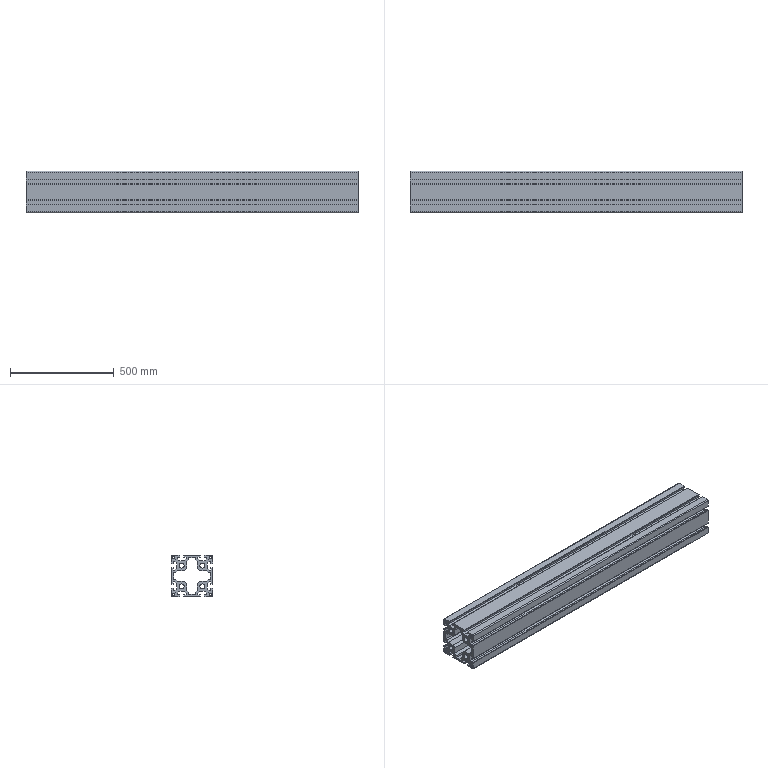Component | SolidWorks | AluminumProfile100x100-1 | 1 solid | 186 faces | box 1600 x 200 x 200 mm | volume 26355047 mm3 | plane 162 | cylinder 24 | commonest cylinder face diameters 12 x12 24 x8 10 x4
build123d program:
from build123d import *

# Parameters (mm, degrees)
SKETCH1_R           = 6
BOSS_EXTRUDE1_DEPTH = 800
SCALE1_SCALE        = 2


with BuildPart() as part:
    # Sketch1 → Boss-Extrude1 (new body)
    with BuildSketch(Plane(origin=(-310, 0, 0), x_dir=(0, -1, 0), z_dir=(-1, 0, 0))):
        with BuildLine():
            Line((45, 19.9), (45, 14))
            Line((45, 14), (41.657, 14))
            Line((41.657, 14), (37.2, 18.457))
            Line((37.2, 18.457), (37.2, 31.543))
            Line((37.2, 31.543), (41.657, 36))
            Line((41.657, 36), (45, 36))
            Line((45, 36), (45, 30.1))
            Line((45, 30.1), (49, 30.1))
            Line((49, 30.1), (49, 31.1))
            Line((49, 31.1), (50, 31.1))
            Line((50, 31.1), (50, 47.5))
            ThreePointArc((50, 47.5), (49.268, 49.268), (47.5, 50))
            Line((47.5, 50), (31.1, 50))
            Line((31.1, 50), (31.1, 49))
            Line((31.1, 49), (30.1, 49))
            Line((30.1, 49), (30.1, 45))
            Line((30.1, 45), (36, 45))
            Line((36, 45), (36, 41.657))
            Line((36, 41.657), (31.543, 37.2))
            Line((31.543, 37.2), (18.457, 37.2))
            Line((18.457, 37.2), (14, 41.657))
            Line((14, 41.657), (14, 45))
            Line((14, 45), (19.9, 45))
            Line((19.9, 45), (19.9, 49))
            Line((19.9, 49), (18.9, 49))
            Line((18.9, 49), (18.9, 50))
            Line((18.9, 50), (-18.9, 50))
            Line((-18.9, 50), (-18.9, 49))
            Line((-18.9, 49), (-19.9, 49))
            Line((-19.9, 49), (-19.9, 45))
            Line((-19.9, 45), (-14, 45))
            Line((-14, 45), (-14, 41.657))
            Line((-14, 41.657), (-18.457, 37.2))
            Line((-18.457, 37.2), (-31.543, 37.2))
            Line((-31.543, 37.2), (-36, 41.657))
            Line((-36, 41.657), (-36, 45))
            Line((-36, 45), (-30.1, 45))
            Line((-30.1, 45), (-30.1, 49))
            Line((-30.1, 49), (-31.1, 49))
            Line((-31.1, 49), (-31.1, 50))
            Line((-31.1, 50), (-47.5, 50))
            ThreePointArc((-47.5, 50), (-49.268, 49.268), (-50, 47.5))
            Line((-50, 47.5), (-50, 31.1))
            Line((-50, 31.1), (-49, 31.1))
            Line((-49, 31.1), (-49, 30.1))
            Line((-49, 30.1), (-45, 30.1))
            Line((-45, 30.1), (-45, 36))
            Line((-45, 36), (-41.657, 36))
            Line((-41.657, 36), (-37.2, 31.543))
            Line((-37.2, 31.543), (-37.2, 18.457))
            Line((-37.2, 18.457), (-41.657, 14))
            Line((-41.657, 14), (-45, 14))
            Line((-45, 14), (-45, 19.9))
            Line((-45, 19.9), (-49, 19.9))
            Line((-49, 19.9), (-49, 18.9))
            Line((-49, 18.9), (-50, 18.9))
            Line((-50, 18.9), (-50, -18.9))
            Line((-50, -18.9), (-49, -18.9))
            Line((-49, -18.9), (-49, -19.9))
            Line((-49, -19.9), (-45, -19.9))
            Line((-45, -19.9), (-45, -14))
            Line((-45, -14), (-41.657, -14))
            Line((-41.657, -14), (-37.2, -18.457))
            Line((-37.2, -18.457), (-37.2, -31.543))
            Line((-37.2, -31.543), (-41.657, -36))
            Line((-41.657, -36), (-45, -36))
            Line((-45, -36), (-45, -30.1))
            Line((-45, -30.1), (-49, -30.1))
            Line((-49, -30.1), (-49, -31.1))
            Line((-49, -31.1), (-50, -31.1))
            Line((-50, -31.1), (-50, -47.5))
            ThreePointArc((-50, -47.5), (-49.268, -49.268), (-47.5, -50))
            Line((-47.5, -50), (-31.1, -50))
            Line((-31.1, -50), (-31.1, -49))
            Line((-31.1, -49), (-30.1, -49))
            Line((-30.1, -49), (-30.1, -45))
            Line((-30.1, -45), (-36, -45))
            Line((-36, -45), (-36, -41.657))
            Line((-36, -41.657), (-31.543, -37.2))
            Line((-31.543, -37.2), (-18.457, -37.2))
            Line((-18.457, -37.2), (-14, -41.657))
            Line((-14, -41.657), (-14, -45))
            Line((-14, -45), (-19.9, -45))
            Line((-19.9, -45), (-19.9, -49))
            Line((-19.9, -49), (-18.9, -49))
            Line((-18.9, -49), (-18.9, -50))
            Line((-18.9, -50), (18.9, -50))
            Line((18.9, -50), (18.9, -49))
            Line((18.9, -49), (19.9, -49))
            Line((19.9, -49), (19.9, -45))
            Line((19.9, -45), (14, -45))
            Line((14, -45), (14, -41.657))
            Line((14, -41.657), (18.457, -37.2))
            Line((18.457, -37.2), (31.543, -37.2))
            Line((31.543, -37.2), (36, -41.657))
            Line((36, -41.657), (36, -45))
            Line((36, -45), (30.1, -45))
            Line((30.1, -45), (30.1, -49))
            Line((30.1, -49), (31.1, -49))
            Line((31.1, -49), (31.1, -50))
            Line((31.1, -50), (47.5, -50))
            ThreePointArc((47.5, -50), (49.268, -49.268), (50, -47.5))
            Line((50, -47.5), (50, -31.1))
            Line((50, -31.1), (49, -31.1))
            Line((49, -31.1), (49, -30.1))
            Line((49, -30.1), (45, -30.1))
            Line((45, -30.1), (45, -36))
            Line((45, -36), (41.657, -36))
            Line((41.657, -36), (37.2, -31.543))
            Line((37.2, -31.543), (37.2, -18.457))
            Line((37.2, -18.457), (41.657, -14))
            Line((41.657, -14), (45, -14))
            Line((45, -14), (45, -19.9))
            Line((45, -19.9), (49, -19.9))
            Line((49, -19.9), (49, -18.9))
            Line((49, -18.9), (50, -18.9))
            Line((50, -18.9), (50, 18.9))
            Line((50, 18.9), (49, 18.9))
            Line((49, 18.9), (49, 19.9))
            Line((49, 19.9), (45, 19.9))
        make_face()
        with Locations(Location((25, 25, 0), (0, 0, 180))):
            Circle(SKETCH1_R, mode=Mode.SUBTRACT)
        with Locations(Location((25, -25, 0), (0, 0, 180))):
            Circle(SKETCH1_R, mode=Mode.SUBTRACT)
        with Locations(Location((-25, 25, 0), (0, 0, 180))):
            Circle(SKETCH1_R, mode=Mode.SUBTRACT)
        with Locations(Location((-25, -25, 0), (0, 0, 180))):
            Circle(SKETCH1_R, mode=Mode.SUBTRACT)
        with BuildLine():
            Line((38.981, -40.678), (40.678, -38.981))
            Line((40.678, -38.981), (42.904, -41.207))
            ThreePointArc((42.904, -41.207), (46.121, -46.121), (41.207, -42.904))
            Line((41.207, -42.904), (38.981, -40.678))
        make_face(mode=Mode.SUBTRACT)
        with BuildLine():
            Line((-40.678, -38.981), (-38.981, -40.678))
            Line((-38.981, -40.678), (-41.207, -42.904))
            ThreePointArc((-41.207, -42.904), (-46.121, -46.121), (-42.904, -41.207))
            Line((-42.904, -41.207), (-40.678, -38.981))
        make_face(mode=Mode.SUBTRACT)
        Polygon((34.372, 12.8), (39.172, 8), (44, 8), (44, -8), (39.172, -8), (34.372, -12.8), (18.8, -12.8), (12.8, -18.8), (12.8, -34.372), (8, -39.172), (8, -44), (-8, -44), (-8, -39.172), (-12.8, -34.372), (-12.8, -18.8), (-18.8, -12.8), (-34.372, -12.8), (-39.172, -8), (-44, -8), (-44, 8), (-39.172, 8), (-34.372, 12.8), (-18.8, 12.8), (-12.8, 18.8), (-12.8, 34.372), (-8, 39.172), (-8, 44), (8, 44), (8, 39.172), (12.8, 34.372), (12.8, 18.8), (18.8, 12.8), align=None, mode=Mode.SUBTRACT)
        with BuildLine():
            Line((42.904, 41.207), (40.678, 38.981))
            Line((40.678, 38.981), (38.981, 40.678))
            Line((38.981, 40.678), (41.207, 42.904))
            ThreePointArc((41.207, 42.904), (46.121, 46.121), (42.904, 41.207))
        make_face(mode=Mode.SUBTRACT)
        with BuildLine():
            Line((-41.207, 42.904), (-38.981, 40.678))
            Line((-38.981, 40.678), (-40.678, 38.981))
            Line((-40.678, 38.981), (-42.904, 41.207))
            ThreePointArc((-42.904, 41.207), (-46.121, 46.121), (-41.207, 42.904))
        make_face(mode=Mode.SUBTRACT)
    extrude(amount=-BOSS_EXTRUDE1_DEPTH)


with BuildPart() as part_1:
    # Scale1: scaled about (90, 0, -0)
    add(part.part.scale(SCALE1_SCALE).moved(Location((-90, 0, 0))))


solid = part_1.part

# Placed as in the assembly
solid = solid.moved(Location((1296, -931, -255), (0, 0, 0)))